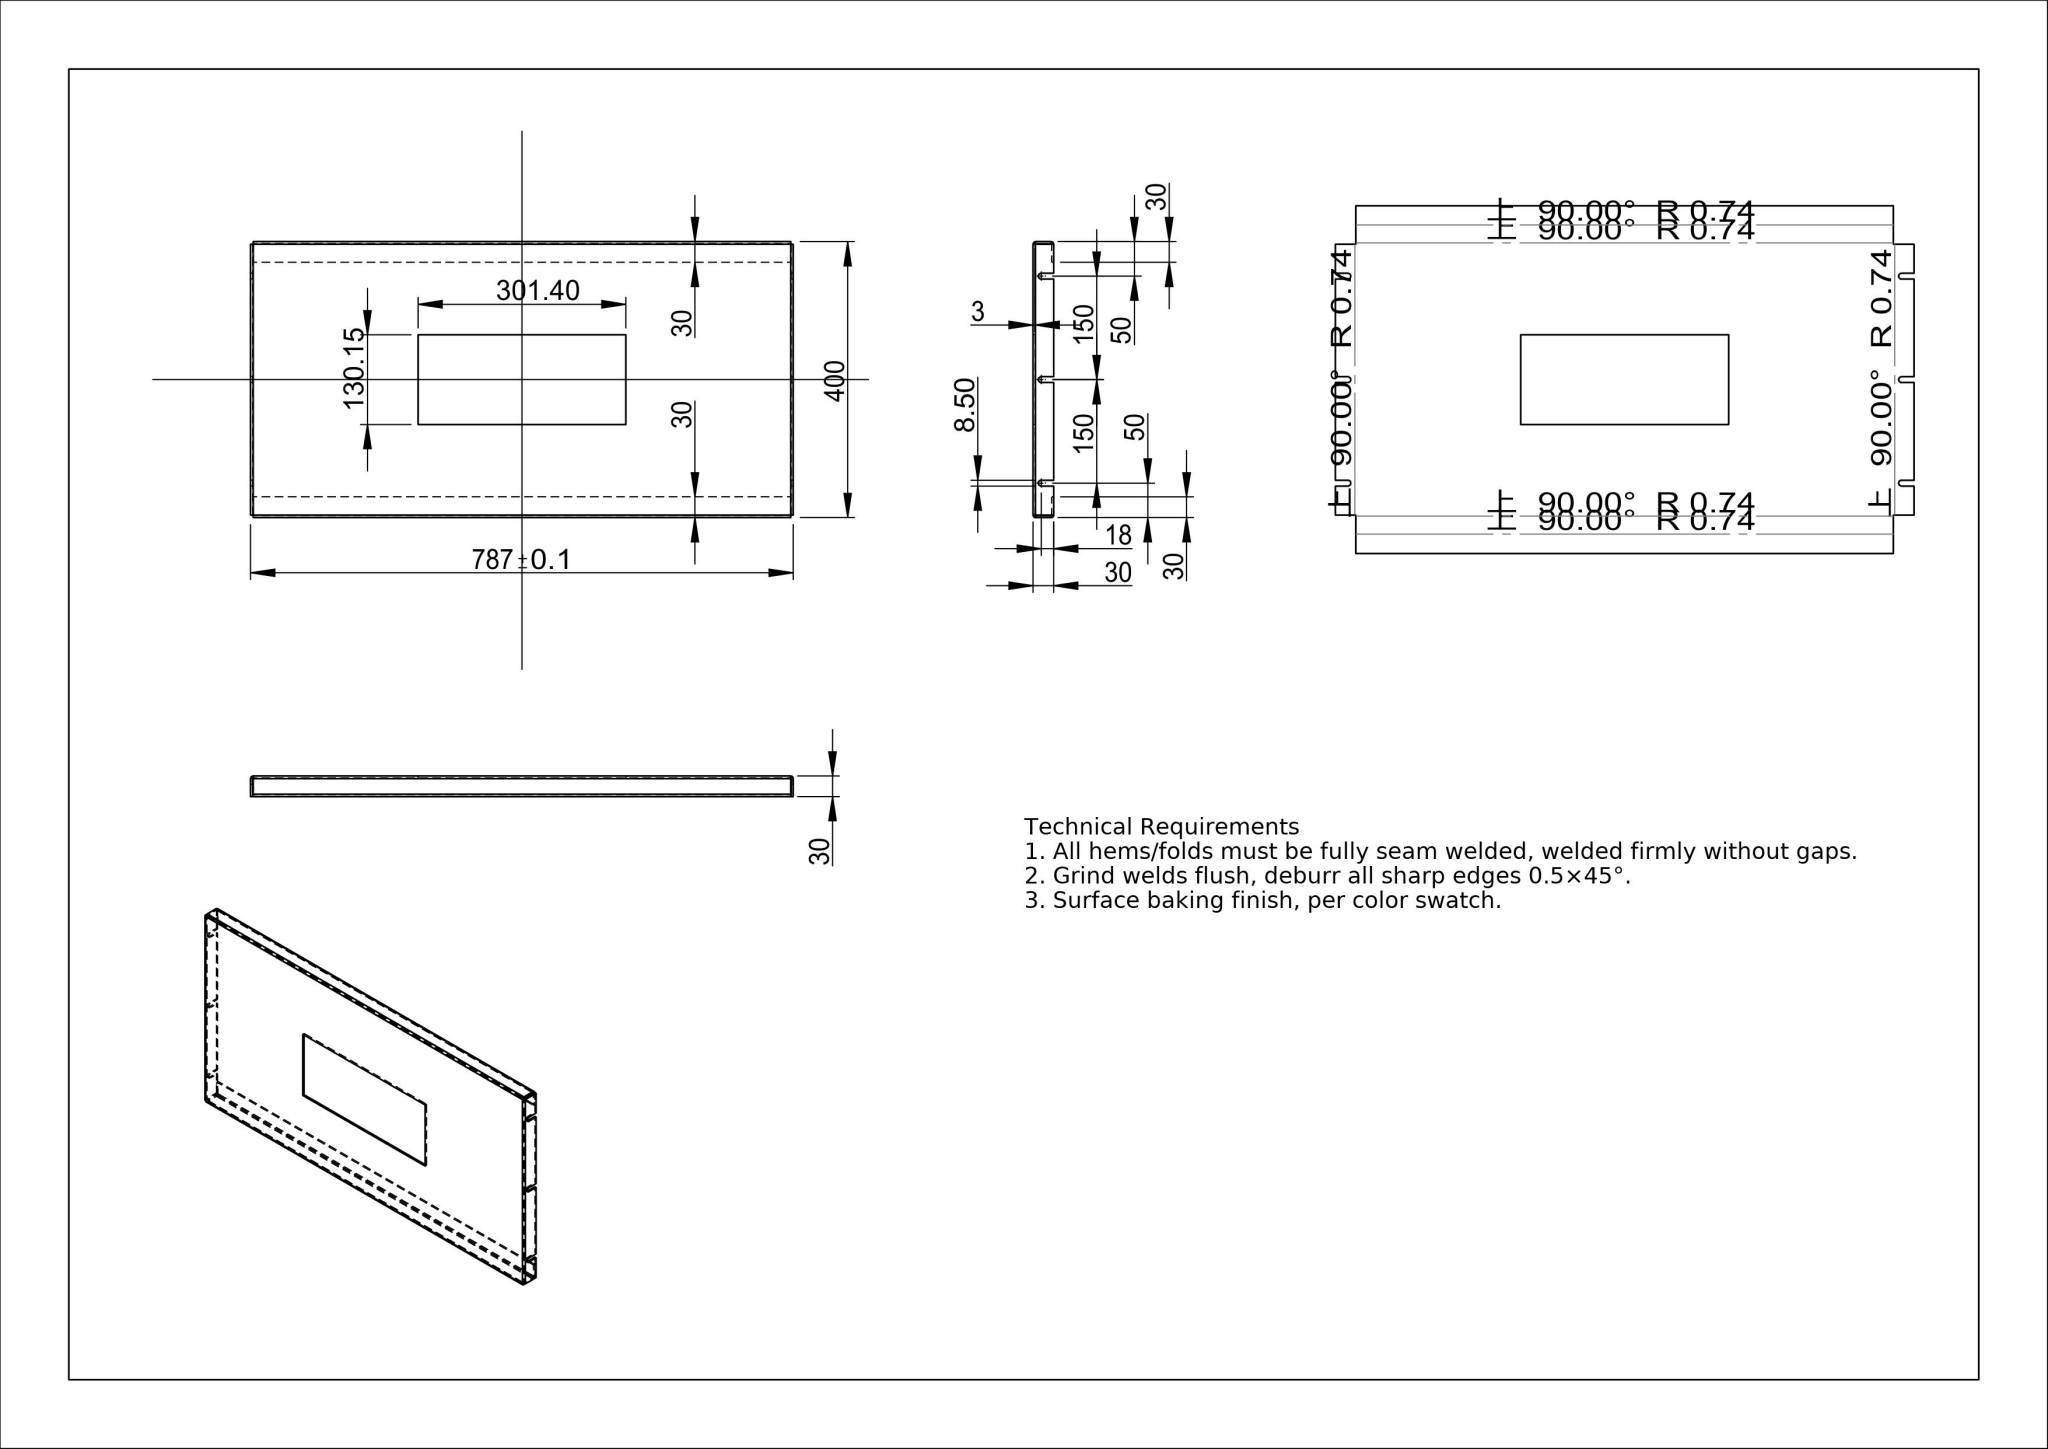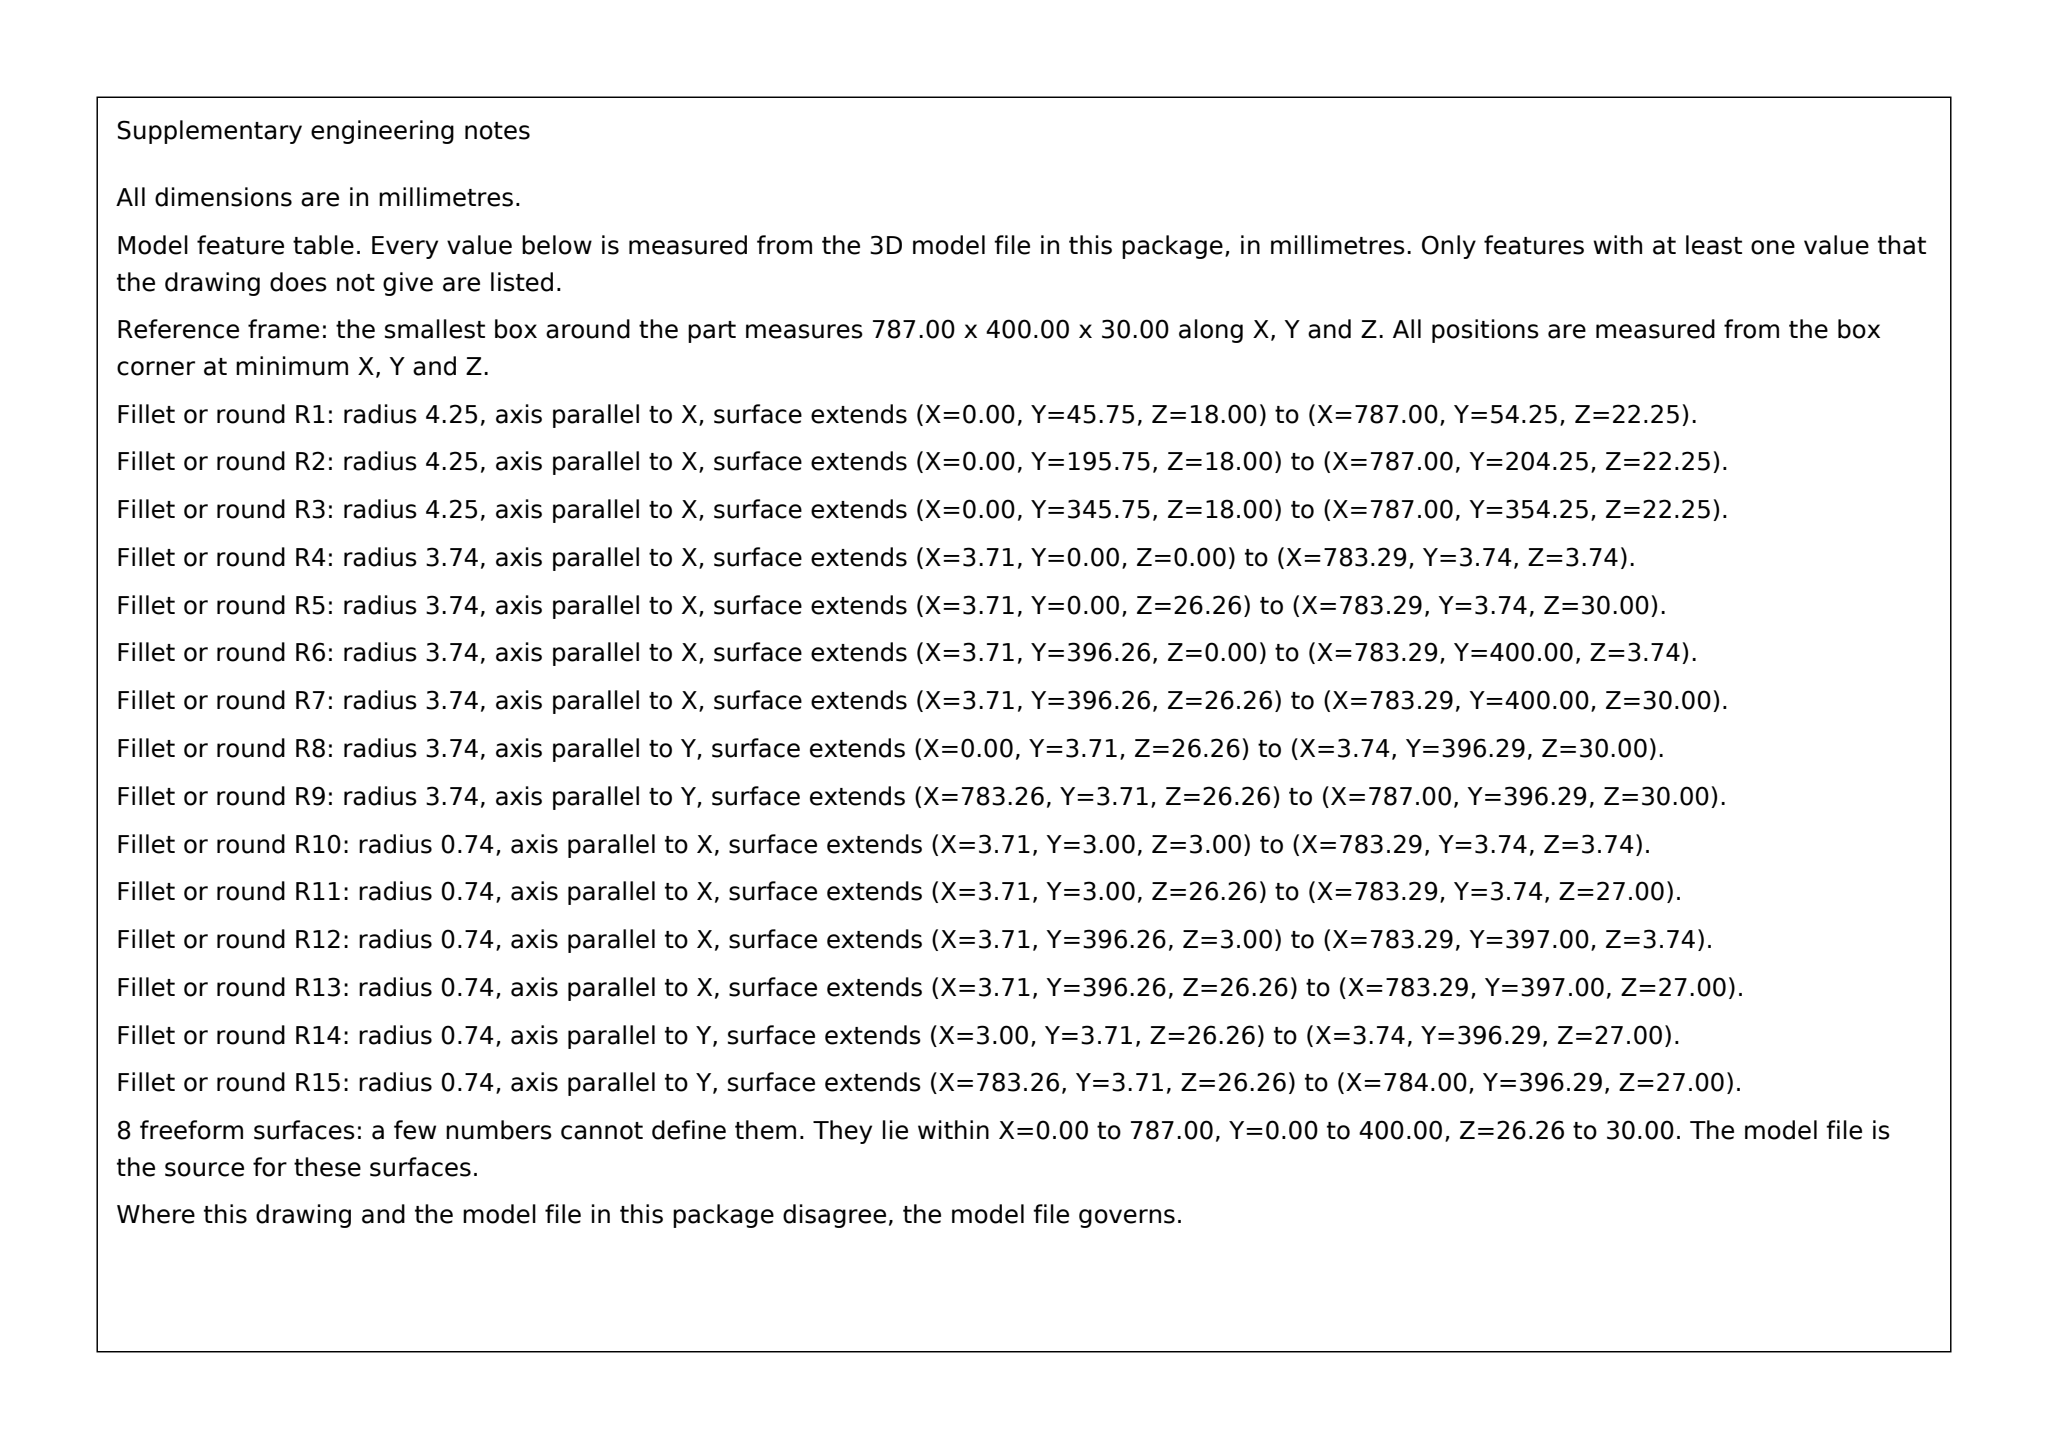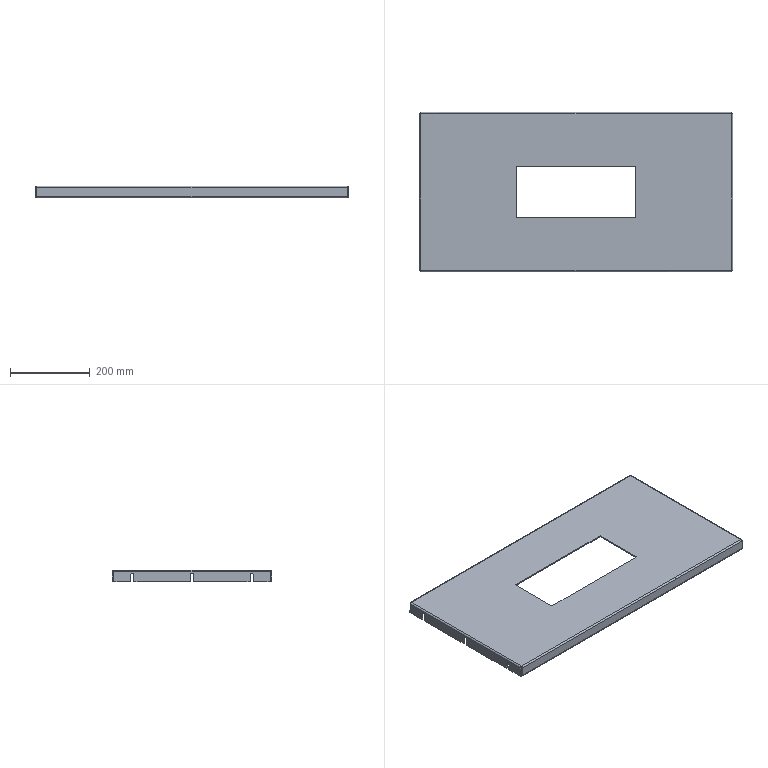Part | SolidWorks | mm | 1 solid | 82 faces | box 787 x 400 x 30 mm | volume 1128228 mm3 | plane 56 | cylinder 18 | spline 8 | commonest cylinder face diameters 7.473 x6 1.473 x6 8.5 x6